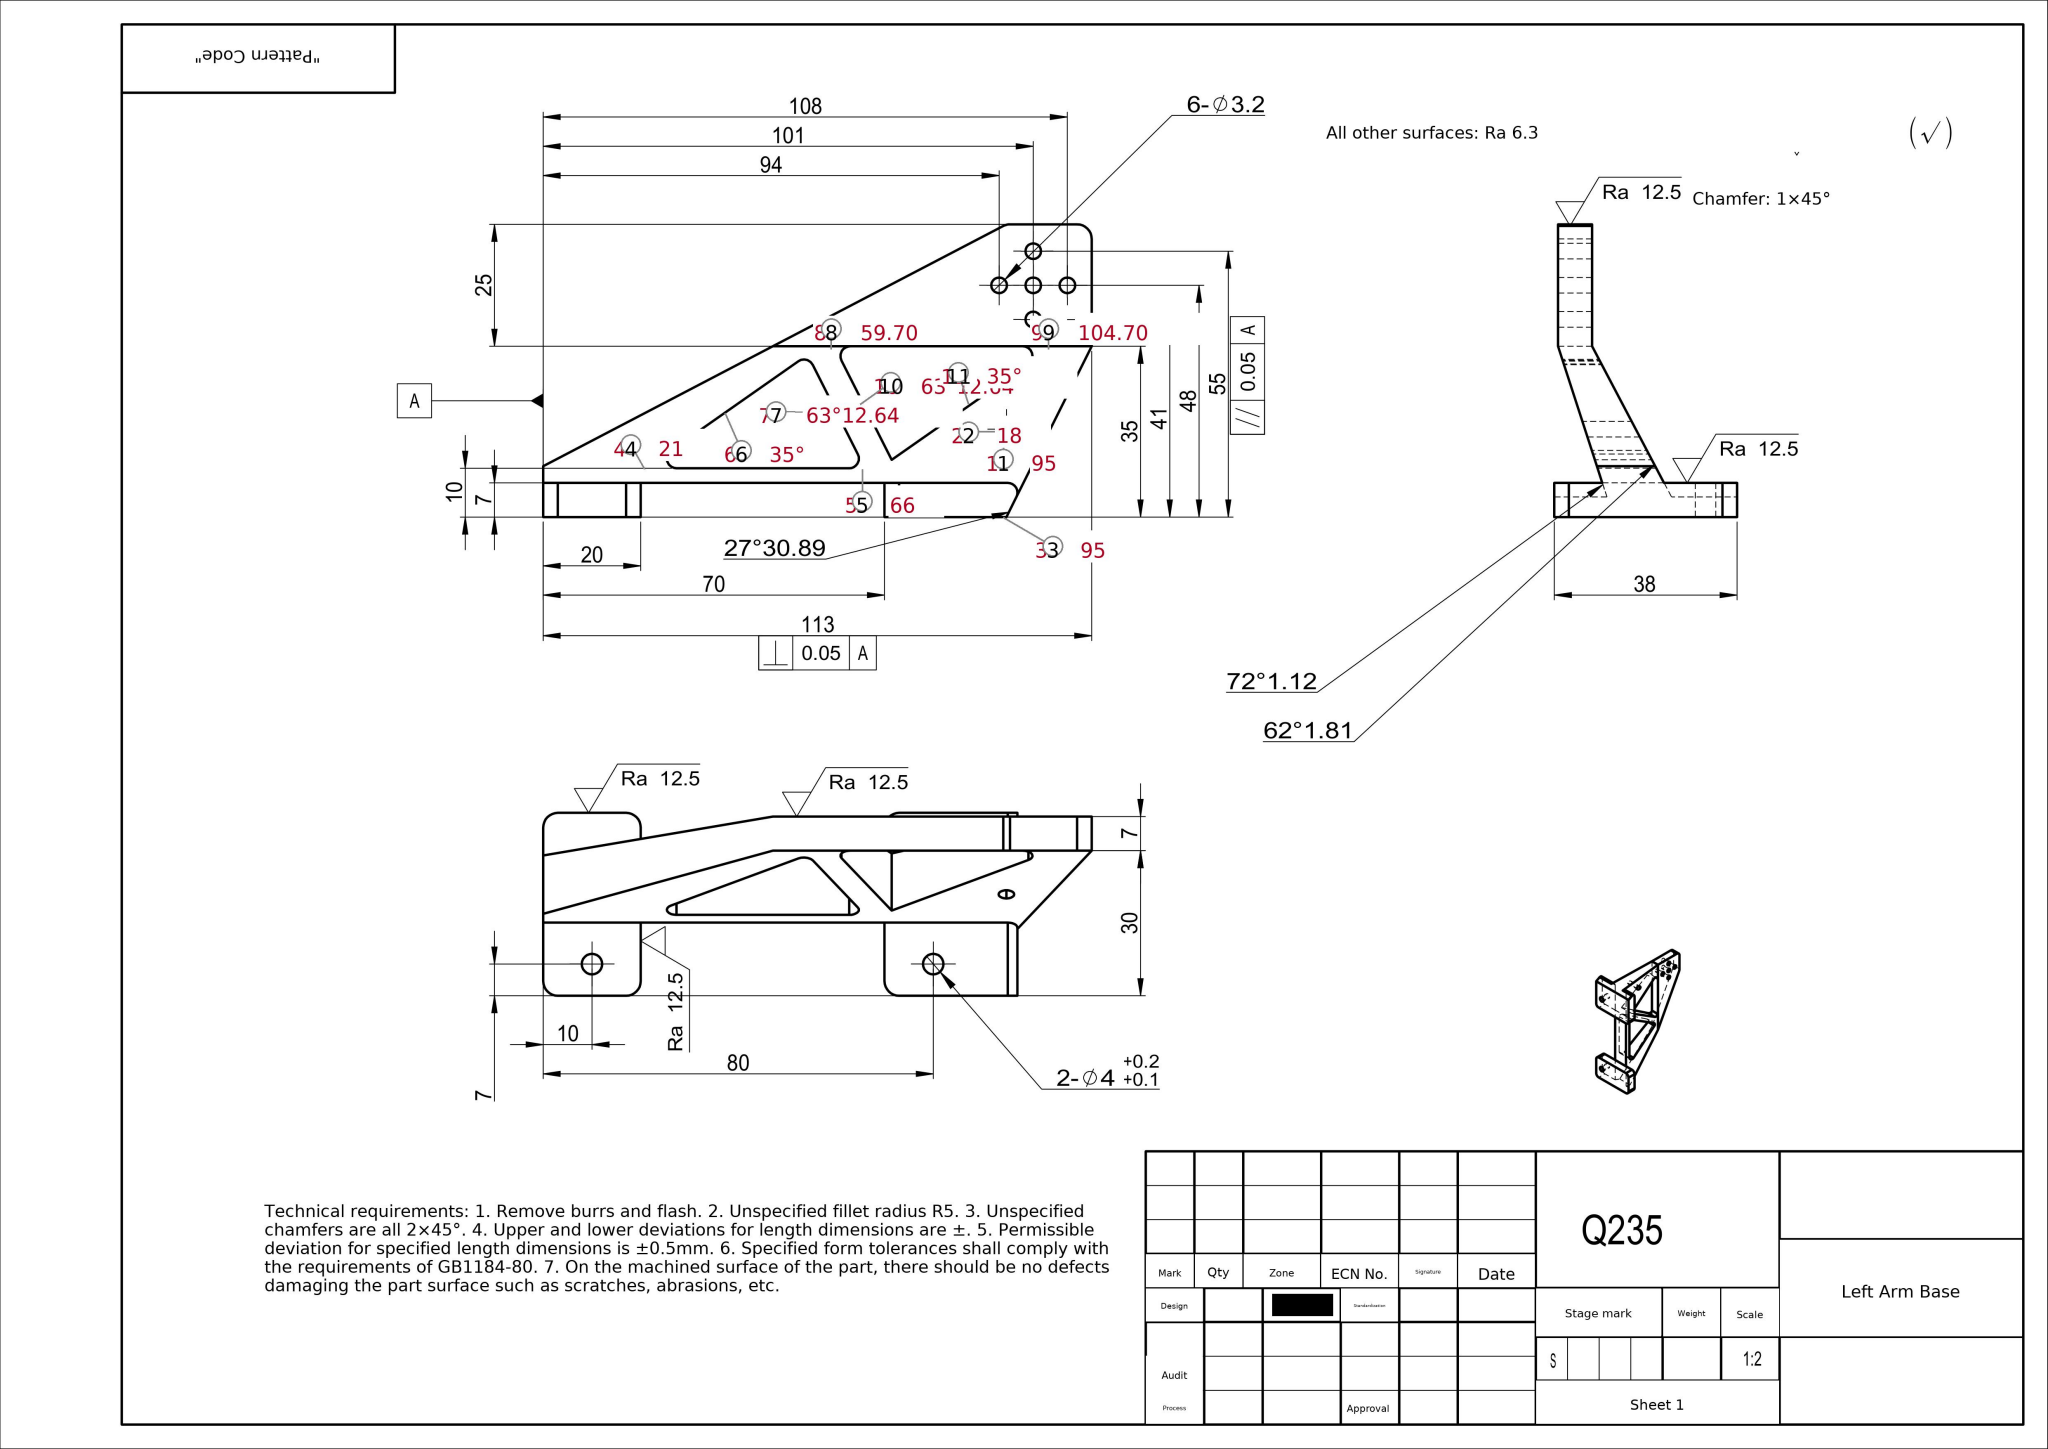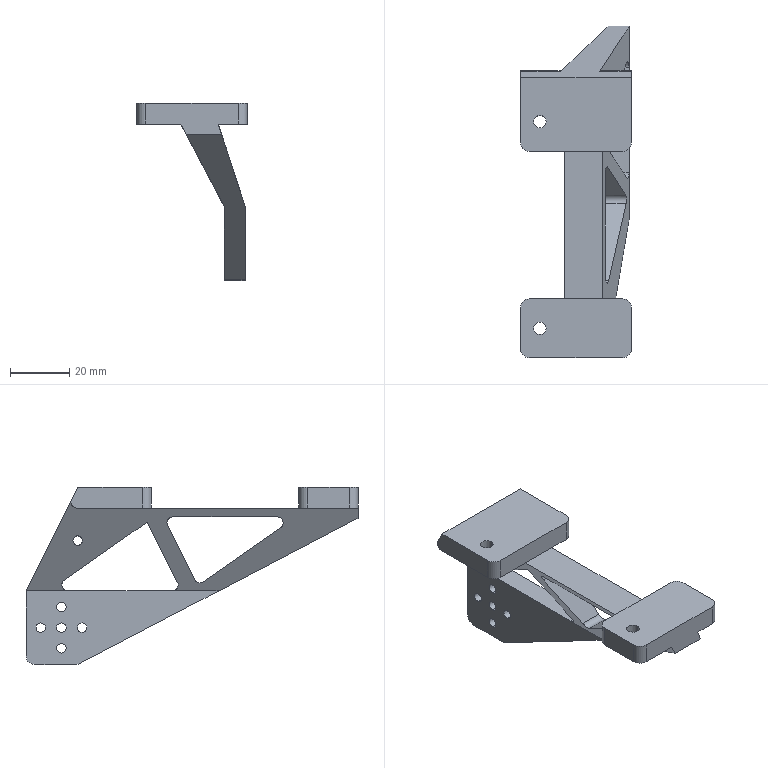Part | SolidWorks | mm | material Q235 | 1 solid | 59 faces | box 37.5 x 112.5 x 60 mm | volume 32875 mm3 | cylinder 31 | plane 28 | commonest cylinder face diameters 3.2 x12 6 x8 4 x7 4.2 x4